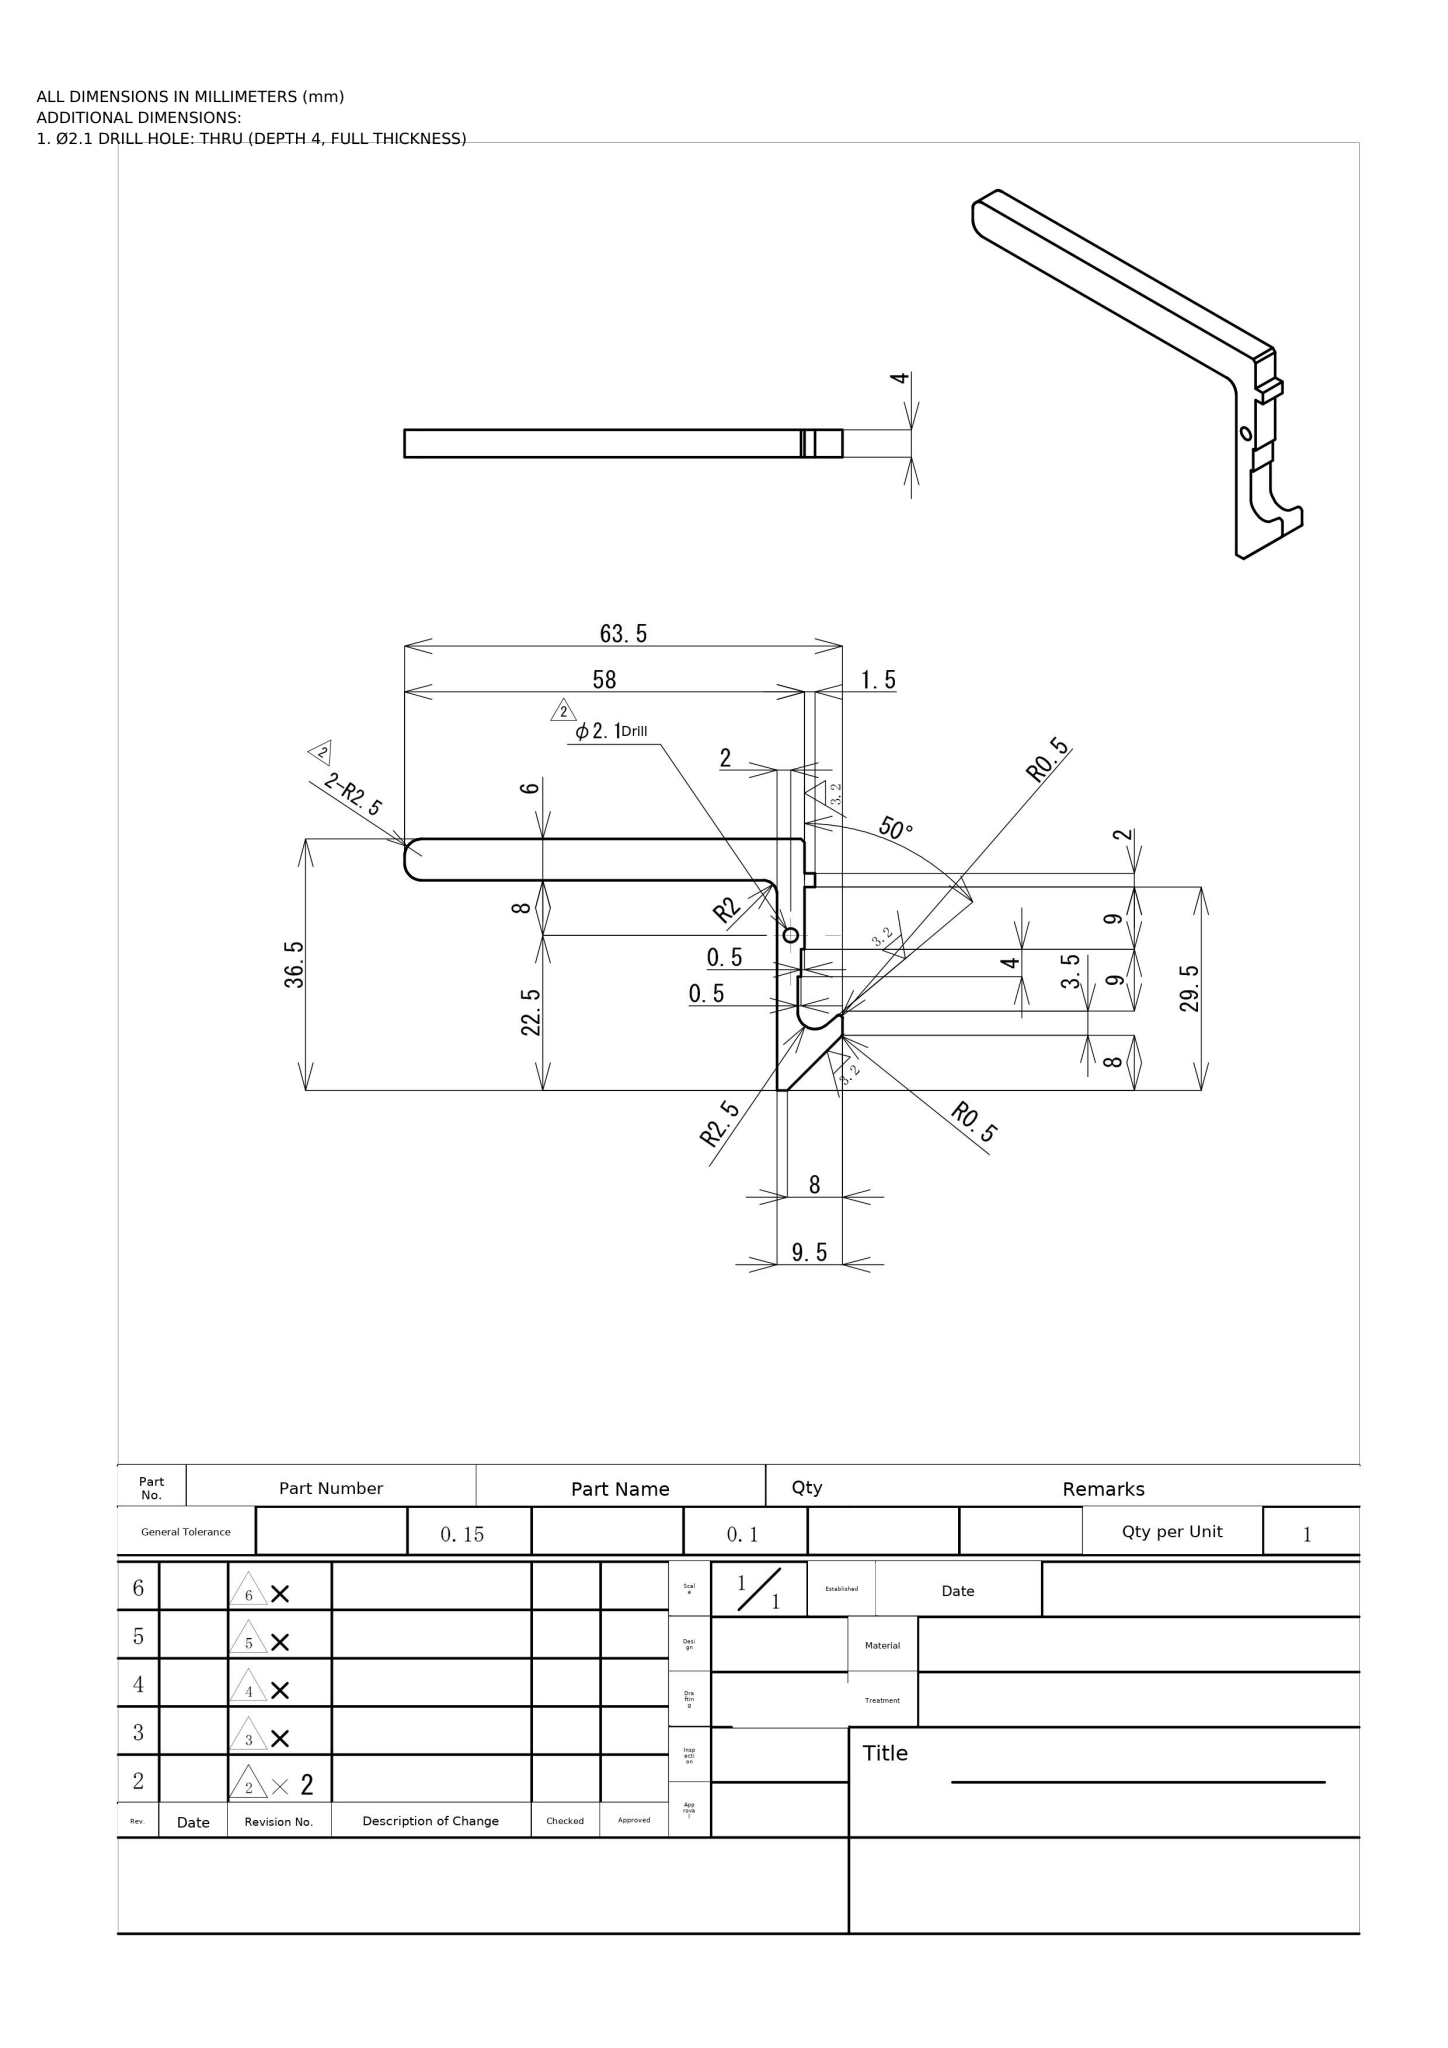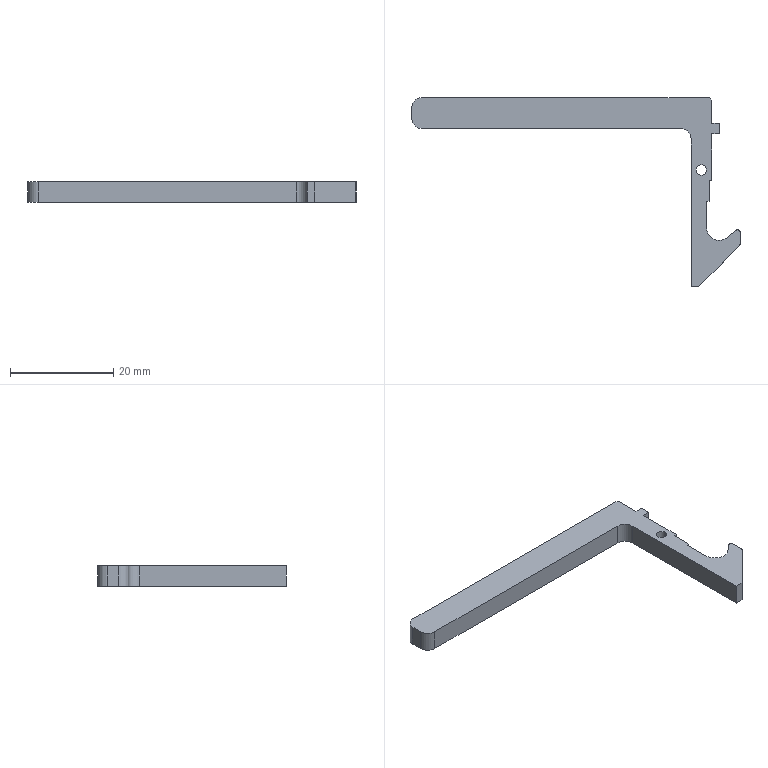Part | NX | mm | 1 solid | 28 faces | box 63.5 x 36.5 x 4 mm | volume 1926 mm3 | plane 20 | cylinder 8 | commonest cylinder face diameters 4 x3 2 x2 1 x2 5 x1